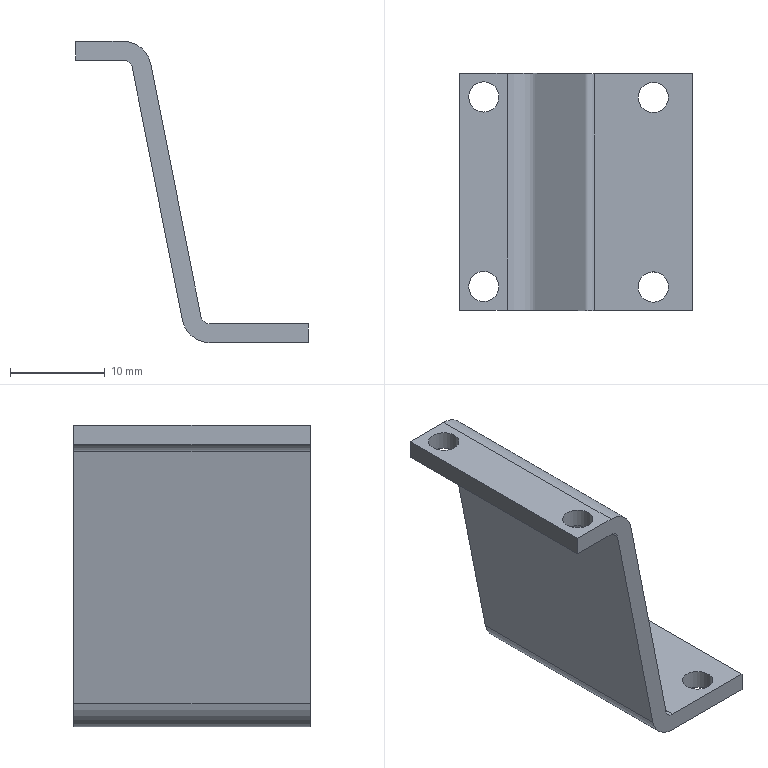Component | NX | BRACKET | 1 solid | 18 faces | volume 2333 mm3 | plane 10 | cylinder 8 | commonest cylinder face diameters 3.2 x4 6 x2 2 x2